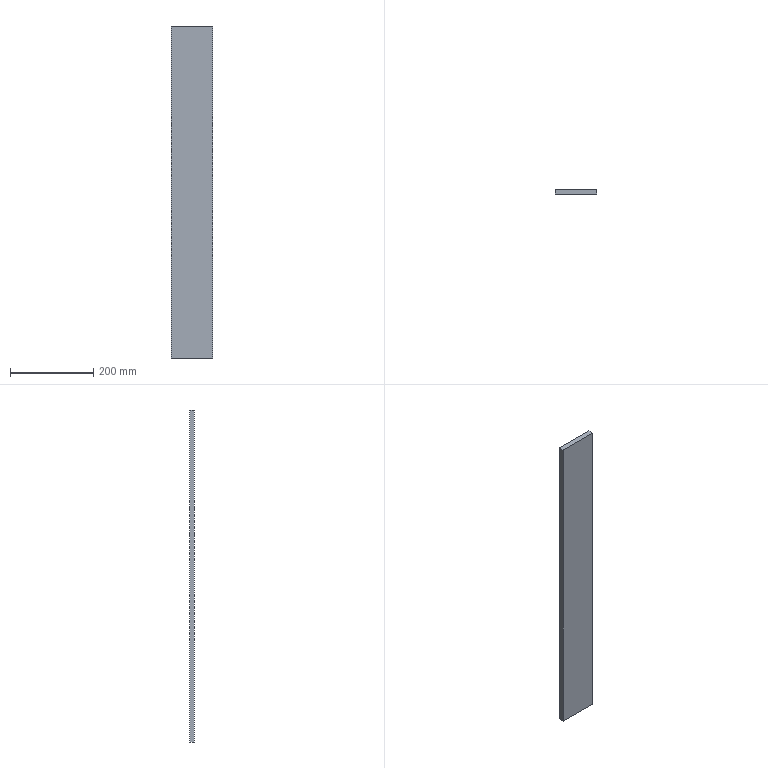Component | NX | CHAPA_LATERAL | 1 solid | 6 faces | box 100 x 12 x 800 mm | volume 960000 mm3 | plane 6
STEP:
#1=CARTESIAN_POINT('',(0.,0.,0.));
#2=DIRECTION('',(0.,0.,1.));
#3=DIRECTION('',(1.,0.,0.));
#4=AXIS2_PLACEMENT_3D('',#1,#2,#3);
#5=CARTESIAN_POINT('',(0.,77.2,800.));
#6=VERTEX_POINT('',#5);
#7=CARTESIAN_POINT('',(0.,77.2,0.));
#8=VERTEX_POINT('',#7);
#9=CARTESIAN_POINT('',(0.,77.2,800.));
#10=DIRECTION('',(0.,0.,-1.));
#11=VECTOR('',#10,1.);
#12=LINE('',#9,#11);
#13=CARTESIAN_POINT('',(0.,65.2,800.));
#14=DIRECTION('',(1.,0.,0.));
#15=DIRECTION('',(0.,0.,-1.));
#16=AXIS2_PLACEMENT_3D('',#13,#14,#15);
#17=PLANE('',#16);
#18=CARTESIAN_POINT('',(0.,12.));
#19=DIRECTION('',(1.,0.));
#20=VECTOR('',#19,1.);
#21=LINE('',#18,#20);
#22=(GEOMETRIC_REPRESENTATION_CONTEXT(2)PARAMETRIC_REPRESENTATION_CONTEXT()REPRESENTATION_CONTEXT('',''));
#23=DEFINITIONAL_REPRESENTATION('',(#21),#22);
#24=PCURVE('',#17,#23);
#25=CARTESIAN_POINT('',(0.,77.2,0.));
#26=DIRECTION('',(0.,-1.,0.));
#27=DIRECTION('',(0.,0.,-1.));
#28=AXIS2_PLACEMENT_3D('',#25,#26,#27);
#29=PLANE('',#28);
#30=CARTESIAN_POINT('',(-800.,-0.));
#31=DIRECTION('',(1.,0.));
#32=VECTOR('',#31,1.);
#33=LINE('',#30,#32);
#34=(GEOMETRIC_REPRESENTATION_CONTEXT(2)PARAMETRIC_REPRESENTATION_CONTEXT()REPRESENTATION_CONTEXT('',''));
#35=DEFINITIONAL_REPRESENTATION('',(#33),#34);
#36=PCURVE('',#29,#35);
#37=SURFACE_CURVE('',#12,(#24,#36),.PCURVE_S1.);
#38=EDGE_CURVE('',#6,#8,#37,.T.);
#39=ORIENTED_EDGE('',*,*,#38,.T.);
#40=CARTESIAN_POINT('',(0.,65.2,0.));
#41=VERTEX_POINT('',#40);
#42=CARTESIAN_POINT('',(0.,65.2,0.));
#43=DIRECTION('',(0.,1.,0.));
#44=VECTOR('',#43,1.);
#45=LINE('',#42,#44);
#46=CARTESIAN_POINT('',(800.,0.));
#47=DIRECTION('',(0.,1.));
#48=VECTOR('',#47,1.);
#49=LINE('',#46,#48);
#50=(GEOMETRIC_REPRESENTATION_CONTEXT(2)PARAMETRIC_REPRESENTATION_CONTEXT()REPRESENTATION_CONTEXT('',''));
#51=DEFINITIONAL_REPRESENTATION('',(#49),#50);
#52=PCURVE('',#17,#51);
#53=CARTESIAN_POINT('',(0.,65.2,0.));
#54=DIRECTION('',(-0.,0.,1.));
#55=DIRECTION('',(1.,0.,0.));
#56=AXIS2_PLACEMENT_3D('',#53,#54,#55);
#57=PLANE('',#56);
#58=CARTESIAN_POINT('',(0.,0.));
#59=DIRECTION('',(0.,1.));
#60=VECTOR('',#59,1.);
#61=LINE('',#58,#60);
#62=(GEOMETRIC_REPRESENTATION_CONTEXT(2)PARAMETRIC_REPRESENTATION_CONTEXT()REPRESENTATION_CONTEXT('',''));
#63=DEFINITIONAL_REPRESENTATION('',(#61),#62);
#64=PCURVE('',#57,#63);
#65=SURFACE_CURVE('',#45,(#52,#64),.PCURVE_S1.);
#66=EDGE_CURVE('',#41,#8,#65,.T.);
#67=ORIENTED_EDGE('',*,*,#66,.F.);
#68=CARTESIAN_POINT('',(0.,65.2,800.));
#69=VERTEX_POINT('',#68);
#70=CARTESIAN_POINT('',(0.,65.2,800.));
#71=DIRECTION('',(0.,0.,-1.));
#72=VECTOR('',#71,1.);
#73=LINE('',#70,#72);
#74=CARTESIAN_POINT('',(0.,0.));
#75=DIRECTION('',(1.,0.));
#76=VECTOR('',#75,1.);
#77=LINE('',#74,#76);
#78=(GEOMETRIC_REPRESENTATION_CONTEXT(2)PARAMETRIC_REPRESENTATION_CONTEXT()REPRESENTATION_CONTEXT('',''));
#79=DEFINITIONAL_REPRESENTATION('',(#77),#78);
#80=PCURVE('',#17,#79);
#81=CARTESIAN_POINT('',(0.,65.2,0.));
#82=DIRECTION('',(0.,-1.,0.));
#83=DIRECTION('',(0.,0.,-1.));
#84=AXIS2_PLACEMENT_3D('',#81,#82,#83);
#85=PLANE('',#84);
#86=CARTESIAN_POINT('',(-800.,-0.));
#87=DIRECTION('',(1.,0.));
#88=VECTOR('',#87,1.);
#89=LINE('',#86,#88);
#90=(GEOMETRIC_REPRESENTATION_CONTEXT(2)PARAMETRIC_REPRESENTATION_CONTEXT()REPRESENTATION_CONTEXT('',''));
#91=DEFINITIONAL_REPRESENTATION('',(#89),#90);
#92=PCURVE('',#85,#91);
#93=SURFACE_CURVE('',#73,(#80,#92),.PCURVE_S1.);
#94=EDGE_CURVE('',#69,#41,#93,.T.);
#95=ORIENTED_EDGE('',*,*,#94,.F.);
#96=CARTESIAN_POINT('',(0.,65.2,800.));
#97=DIRECTION('',(0.,1.,0.));
#98=VECTOR('',#97,1.);
#99=LINE('',#96,#98);
#100=CARTESIAN_POINT('',(0.,0.));
#101=DIRECTION('',(0.,1.));
#102=VECTOR('',#101,1.);
#103=LINE('',#100,#102);
#104=(GEOMETRIC_REPRESENTATION_CONTEXT(2)PARAMETRIC_REPRESENTATION_CONTEXT()REPRESENTATION_CONTEXT('',''));
#105=DEFINITIONAL_REPRESENTATION('',(#103),#104);
#106=PCURVE('',#17,#105);
#107=CARTESIAN_POINT('',(100.,65.2,800.));
#108=DIRECTION('',(0.,0.,-1.));
#109=DIRECTION('',(-1.,0.,0.));
#110=AXIS2_PLACEMENT_3D('',#107,#108,#109);
#111=PLANE('',#110);
#112=CARTESIAN_POINT('',(100.,0.));
#113=DIRECTION('',(0.,1.));
#114=VECTOR('',#113,1.);
#115=LINE('',#112,#114);
#116=(GEOMETRIC_REPRESENTATION_CONTEXT(2)PARAMETRIC_REPRESENTATION_CONTEXT()REPRESENTATION_CONTEXT('',''));
#117=DEFINITIONAL_REPRESENTATION('',(#115),#116);
#118=PCURVE('',#111,#117);
#119=SURFACE_CURVE('',#99,(#106,#118),.PCURVE_S1.);
#120=EDGE_CURVE('',#69,#6,#119,.T.);
#121=ORIENTED_EDGE('',*,*,#120,.T.);
#122=EDGE_LOOP('',(#39,#67,#95,#121));
#123=FACE_BOUND('',#122,.T.);
#124=ADVANCED_FACE('',(#123),#17,.F.);
#125=CARTESIAN_POINT('',(100.,77.2,0.));
#126=VERTEX_POINT('',#125);
#127=CARTESIAN_POINT('',(0.,77.2,0.));
#128=DIRECTION('',(1.,0.,0.));
#129=VECTOR('',#128,1.);
#130=LINE('',#127,#129);
#131=CARTESIAN_POINT('',(0.,12.));
#132=DIRECTION('',(1.,0.));
#133=VECTOR('',#132,1.);
#134=LINE('',#131,#133);
#135=(GEOMETRIC_REPRESENTATION_CONTEXT(2)PARAMETRIC_REPRESENTATION_CONTEXT()REPRESENTATION_CONTEXT('',''));
#136=DEFINITIONAL_REPRESENTATION('',(#134),#135);
#137=PCURVE('',#57,#136);
#138=CARTESIAN_POINT('',(0.,0.));
#139=DIRECTION('',(-0.,1.));
#140=VECTOR('',#139,1.);
#141=LINE('',#138,#140);
#142=(GEOMETRIC_REPRESENTATION_CONTEXT(2)PARAMETRIC_REPRESENTATION_CONTEXT()REPRESENTATION_CONTEXT('',''));
#143=DEFINITIONAL_REPRESENTATION('',(#141),#142);
#144=PCURVE('',#29,#143);
#145=SURFACE_CURVE('',#130,(#137,#144),.PCURVE_S1.);
#146=EDGE_CURVE('',#8,#126,#145,.T.);
#147=ORIENTED_EDGE('',*,*,#146,.T.);
#148=CARTESIAN_POINT('',(100.,65.2,0.));
#149=VERTEX_POINT('',#148);
#150=CARTESIAN_POINT('',(100.,65.2,0.));
#151=DIRECTION('',(0.,1.,0.));
#152=VECTOR('',#151,1.);
#153=LINE('',#150,#152);
#154=CARTESIAN_POINT('',(100.,0.));
#155=DIRECTION('',(0.,1.));
#156=VECTOR('',#155,1.);
#157=LINE('',#154,#156);
#158=(GEOMETRIC_REPRESENTATION_CONTEXT(2)PARAMETRIC_REPRESENTATION_CONTEXT()REPRESENTATION_CONTEXT('',''));
#159=DEFINITIONAL_REPRESENTATION('',(#157),#158);
#160=PCURVE('',#57,#159);
#161=CARTESIAN_POINT('',(100.,65.2,0.));
#162=DIRECTION('',(-1.,0.,-0.));
#163=DIRECTION('',(-0.,0.,1.));
#164=AXIS2_PLACEMENT_3D('',#161,#162,#163);
#165=PLANE('',#164);
#166=CARTESIAN_POINT('',(0.,0.));
#167=DIRECTION('',(0.,1.));
#168=VECTOR('',#167,1.);
#169=LINE('',#166,#168);
#170=(GEOMETRIC_REPRESENTATION_CONTEXT(2)PARAMETRIC_REPRESENTATION_CONTEXT()REPRESENTATION_CONTEXT('',''));
#171=DEFINITIONAL_REPRESENTATION('',(#169),#170);
#172=PCURVE('',#165,#171);
#173=SURFACE_CURVE('',#153,(#160,#172),.PCURVE_S1.);
#174=EDGE_CURVE('',#149,#126,#173,.T.);
#175=ORIENTED_EDGE('',*,*,#174,.F.);
#176=CARTESIAN_POINT('',(0.,65.2,0.));
#177=DIRECTION('',(1.,0.,0.));
#178=VECTOR('',#177,1.);
#179=LINE('',#176,#178);
#180=CARTESIAN_POINT('',(0.,0.));
#181=DIRECTION('',(1.,0.));
#182=VECTOR('',#181,1.);
#183=LINE('',#180,#182);
#184=(GEOMETRIC_REPRESENTATION_CONTEXT(2)PARAMETRIC_REPRESENTATION_CONTEXT()REPRESENTATION_CONTEXT('',''));
#185=DEFINITIONAL_REPRESENTATION('',(#183),#184);
#186=PCURVE('',#57,#185);
#187=CARTESIAN_POINT('',(0.,0.));
#188=DIRECTION('',(-0.,1.));
#189=VECTOR('',#188,1.);
#190=LINE('',#187,#189);
#191=(GEOMETRIC_REPRESENTATION_CONTEXT(2)PARAMETRIC_REPRESENTATION_CONTEXT()REPRESENTATION_CONTEXT('',''));
#192=DEFINITIONAL_REPRESENTATION('',(#190),#191);
#193=PCURVE('',#85,#192);
#194=SURFACE_CURVE('',#179,(#186,#193),.PCURVE_S1.);
#195=EDGE_CURVE('',#41,#149,#194,.T.);
#196=ORIENTED_EDGE('',*,*,#195,.F.);
#197=ORIENTED_EDGE('',*,*,#66,.T.);
#198=EDGE_LOOP('',(#147,#175,#196,#197));
#199=FACE_BOUND('',#198,.T.);
#200=ADVANCED_FACE('',(#199),#57,.F.);
#201=CARTESIAN_POINT('',(100.,77.2,800.));
#202=VERTEX_POINT('',#201);
#203=CARTESIAN_POINT('',(100.,77.2,0.));
#204=DIRECTION('',(-0.,0.,1.));
#205=VECTOR('',#204,1.);
#206=LINE('',#203,#205);
#207=CARTESIAN_POINT('',(0.,12.));
#208=DIRECTION('',(1.,0.));
#209=VECTOR('',#208,1.);
#210=LINE('',#207,#209);
#211=(GEOMETRIC_REPRESENTATION_CONTEXT(2)PARAMETRIC_REPRESENTATION_CONTEXT()REPRESENTATION_CONTEXT('',''));
#212=DEFINITIONAL_REPRESENTATION('',(#210),#211);
#213=PCURVE('',#165,#212);
#214=CARTESIAN_POINT('',(0.,100.));
#215=DIRECTION('',(-1.,-0.));
#216=VECTOR('',#215,1.);
#217=LINE('',#214,#216);
#218=(GEOMETRIC_REPRESENTATION_CONTEXT(2)PARAMETRIC_REPRESENTATION_CONTEXT()REPRESENTATION_CONTEXT('',''));
#219=DEFINITIONAL_REPRESENTATION('',(#217),#218);
#220=PCURVE('',#29,#219);
#221=SURFACE_CURVE('',#206,(#213,#220),.PCURVE_S1.);
#222=EDGE_CURVE('',#126,#202,#221,.T.);
#223=ORIENTED_EDGE('',*,*,#222,.T.);
#224=CARTESIAN_POINT('',(100.,65.2,800.));
#225=VERTEX_POINT('',#224);
#226=CARTESIAN_POINT('',(100.,65.2,800.));
#227=DIRECTION('',(0.,1.,0.));
#228=VECTOR('',#227,1.);
#229=LINE('',#226,#228);
#230=CARTESIAN_POINT('',(800.,0.));
#231=DIRECTION('',(0.,1.));
#232=VECTOR('',#231,1.);
#233=LINE('',#230,#232);
#234=(GEOMETRIC_REPRESENTATION_CONTEXT(2)PARAMETRIC_REPRESENTATION_CONTEXT()REPRESENTATION_CONTEXT('',''));
#235=DEFINITIONAL_REPRESENTATION('',(#233),#234);
#236=PCURVE('',#165,#235);
#237=CARTESIAN_POINT('',(0.,0.));
#238=DIRECTION('',(0.,1.));
#239=VECTOR('',#238,1.);
#240=LINE('',#237,#239);
#241=(GEOMETRIC_REPRESENTATION_CONTEXT(2)PARAMETRIC_REPRESENTATION_CONTEXT()REPRESENTATION_CONTEXT('',''));
#242=DEFINITIONAL_REPRESENTATION('',(#240),#241);
#243=PCURVE('',#111,#242);
#244=SURFACE_CURVE('',#229,(#236,#243),.PCURVE_S1.);
#245=EDGE_CURVE('',#225,#202,#244,.T.);
#246=ORIENTED_EDGE('',*,*,#245,.F.);
#247=CARTESIAN_POINT('',(100.,65.2,0.));
#248=DIRECTION('',(-0.,0.,1.));
#249=VECTOR('',#248,1.);
#250=LINE('',#247,#249);
#251=CARTESIAN_POINT('',(0.,0.));
#252=DIRECTION('',(1.,0.));
#253=VECTOR('',#252,1.);
#254=LINE('',#251,#253);
#255=(GEOMETRIC_REPRESENTATION_CONTEXT(2)PARAMETRIC_REPRESENTATION_CONTEXT()REPRESENTATION_CONTEXT('',''));
#256=DEFINITIONAL_REPRESENTATION('',(#254),#255);
#257=PCURVE('',#165,#256);
#258=CARTESIAN_POINT('',(0.,100.));
#259=DIRECTION('',(-1.,-0.));
#260=VECTOR('',#259,1.);
#261=LINE('',#258,#260);
#262=(GEOMETRIC_REPRESENTATION_CONTEXT(2)PARAMETRIC_REPRESENTATION_CONTEXT()REPRESENTATION_CONTEXT('',''));
#263=DEFINITIONAL_REPRESENTATION('',(#261),#262);
#264=PCURVE('',#85,#263);
#265=SURFACE_CURVE('',#250,(#257,#264),.PCURVE_S1.);
#266=EDGE_CURVE('',#149,#225,#265,.T.);
#267=ORIENTED_EDGE('',*,*,#266,.F.);
#268=ORIENTED_EDGE('',*,*,#174,.T.);
#269=EDGE_LOOP('',(#223,#246,#267,#268));
#270=FACE_BOUND('',#269,.T.);
#271=ADVANCED_FACE('',(#270),#165,.F.);
#272=CARTESIAN_POINT('',(100.,77.2,800.));
#273=DIRECTION('',(-1.,0.,0.));
#274=VECTOR('',#273,1.);
#275=LINE('',#272,#274);
#276=CARTESIAN_POINT('',(0.,12.));
#277=DIRECTION('',(1.,0.));
#278=VECTOR('',#277,1.);
#279=LINE('',#276,#278);
#280=(GEOMETRIC_REPRESENTATION_CONTEXT(2)PARAMETRIC_REPRESENTATION_CONTEXT()REPRESENTATION_CONTEXT('',''));
#281=DEFINITIONAL_REPRESENTATION('',(#279),#280);
#282=PCURVE('',#111,#281);
#283=CARTESIAN_POINT('',(-800.,100.));
#284=DIRECTION('',(0.,-1.));
#285=VECTOR('',#284,1.);
#286=LINE('',#283,#285);
#287=(GEOMETRIC_REPRESENTATION_CONTEXT(2)PARAMETRIC_REPRESENTATION_CONTEXT()REPRESENTATION_CONTEXT('',''));
#288=DEFINITIONAL_REPRESENTATION('',(#286),#287);
#289=PCURVE('',#29,#288);
#290=SURFACE_CURVE('',#275,(#282,#289),.PCURVE_S1.);
#291=EDGE_CURVE('',#202,#6,#290,.T.);
#292=ORIENTED_EDGE('',*,*,#291,.T.);
#293=ORIENTED_EDGE('',*,*,#120,.F.);
#294=CARTESIAN_POINT('',(100.,65.2,800.));
#295=DIRECTION('',(-1.,0.,0.));
#296=VECTOR('',#295,1.);
#297=LINE('',#294,#296);
#298=CARTESIAN_POINT('',(0.,0.));
#299=DIRECTION('',(1.,0.));
#300=VECTOR('',#299,1.);
#301=LINE('',#298,#300);
#302=(GEOMETRIC_REPRESENTATION_CONTEXT(2)PARAMETRIC_REPRESENTATION_CONTEXT()REPRESENTATION_CONTEXT('',''));
#303=DEFINITIONAL_REPRESENTATION('',(#301),#302);
#304=PCURVE('',#111,#303);
#305=CARTESIAN_POINT('',(-800.,100.));
#306=DIRECTION('',(0.,-1.));
#307=VECTOR('',#306,1.);
#308=LINE('',#305,#307);
#309=(GEOMETRIC_REPRESENTATION_CONTEXT(2)PARAMETRIC_REPRESENTATION_CONTEXT()REPRESENTATION_CONTEXT('',''));
#310=DEFINITIONAL_REPRESENTATION('',(#308),#309);
#311=PCURVE('',#85,#310);
#312=SURFACE_CURVE('',#297,(#304,#311),.PCURVE_S1.);
#313=EDGE_CURVE('',#225,#69,#312,.T.);
#314=ORIENTED_EDGE('',*,*,#313,.F.);
#315=ORIENTED_EDGE('',*,*,#245,.T.);
#316=EDGE_LOOP('',(#292,#293,#314,#315));
#317=FACE_BOUND('',#316,.T.);
#318=ADVANCED_FACE('',(#317),#111,.F.);
#319=ORIENTED_EDGE('',*,*,#94,.T.);
#320=ORIENTED_EDGE('',*,*,#195,.T.);
#321=ORIENTED_EDGE('',*,*,#266,.T.);
#322=ORIENTED_EDGE('',*,*,#313,.T.);
#323=EDGE_LOOP('',(#319,#320,#321,#322));
#324=FACE_BOUND('',#323,.T.);
#325=ADVANCED_FACE('',(#324),#85,.T.);
#326=ORIENTED_EDGE('',*,*,#38,.F.);
#327=ORIENTED_EDGE('',*,*,#291,.F.);
#328=ORIENTED_EDGE('',*,*,#222,.F.);
#329=ORIENTED_EDGE('',*,*,#146,.F.);
#330=EDGE_LOOP('',(#326,#327,#328,#329));
#331=FACE_BOUND('',#330,.T.);
#332=ADVANCED_FACE('',(#331),#29,.F.);
#333=CLOSED_SHELL('',(#124,#200,#271,#318,#325,#332));
#334=MANIFOLD_SOLID_BREP('',#333);
#335=(LENGTH_UNIT()NAMED_UNIT(*)SI_UNIT(.MILLI.,.METRE.));
#336=UNCERTAINTY_MEASURE_WITH_UNIT(LENGTH_MEASURE(0.0000001),#335,'','');
#337=(NAMED_UNIT(*)PLANE_ANGLE_UNIT()SI_UNIT($,.RADIAN.));
#338=(NAMED_UNIT(*)SI_UNIT($,.STERADIAN.)SOLID_ANGLE_UNIT());
#339=(GEOMETRIC_REPRESENTATION_CONTEXT(3)GLOBAL_UNCERTAINTY_ASSIGNED_CONTEXT((#336))GLOBAL_UNIT_ASSIGNED_CONTEXT((#335,#337,#338))REPRESENTATION_CONTEXT('',''));
#340=ADVANCED_BREP_SHAPE_REPRESENTATION('',(#4,#334),#339);